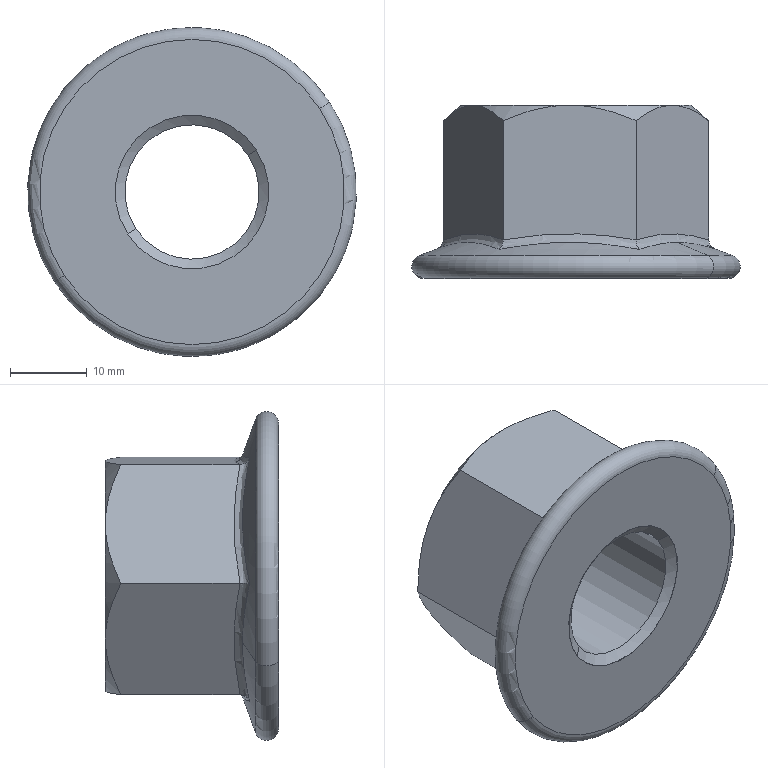Component | SolidWorks | hex flange nut gradea_iso-3 | 1 solid | 32 faces | volume 14336 mm3 | cone 12 | plane 8 | spline 6 | cylinder 4 | torus 2 | commonest cylinder face diameters 20 x2 17.5 x2